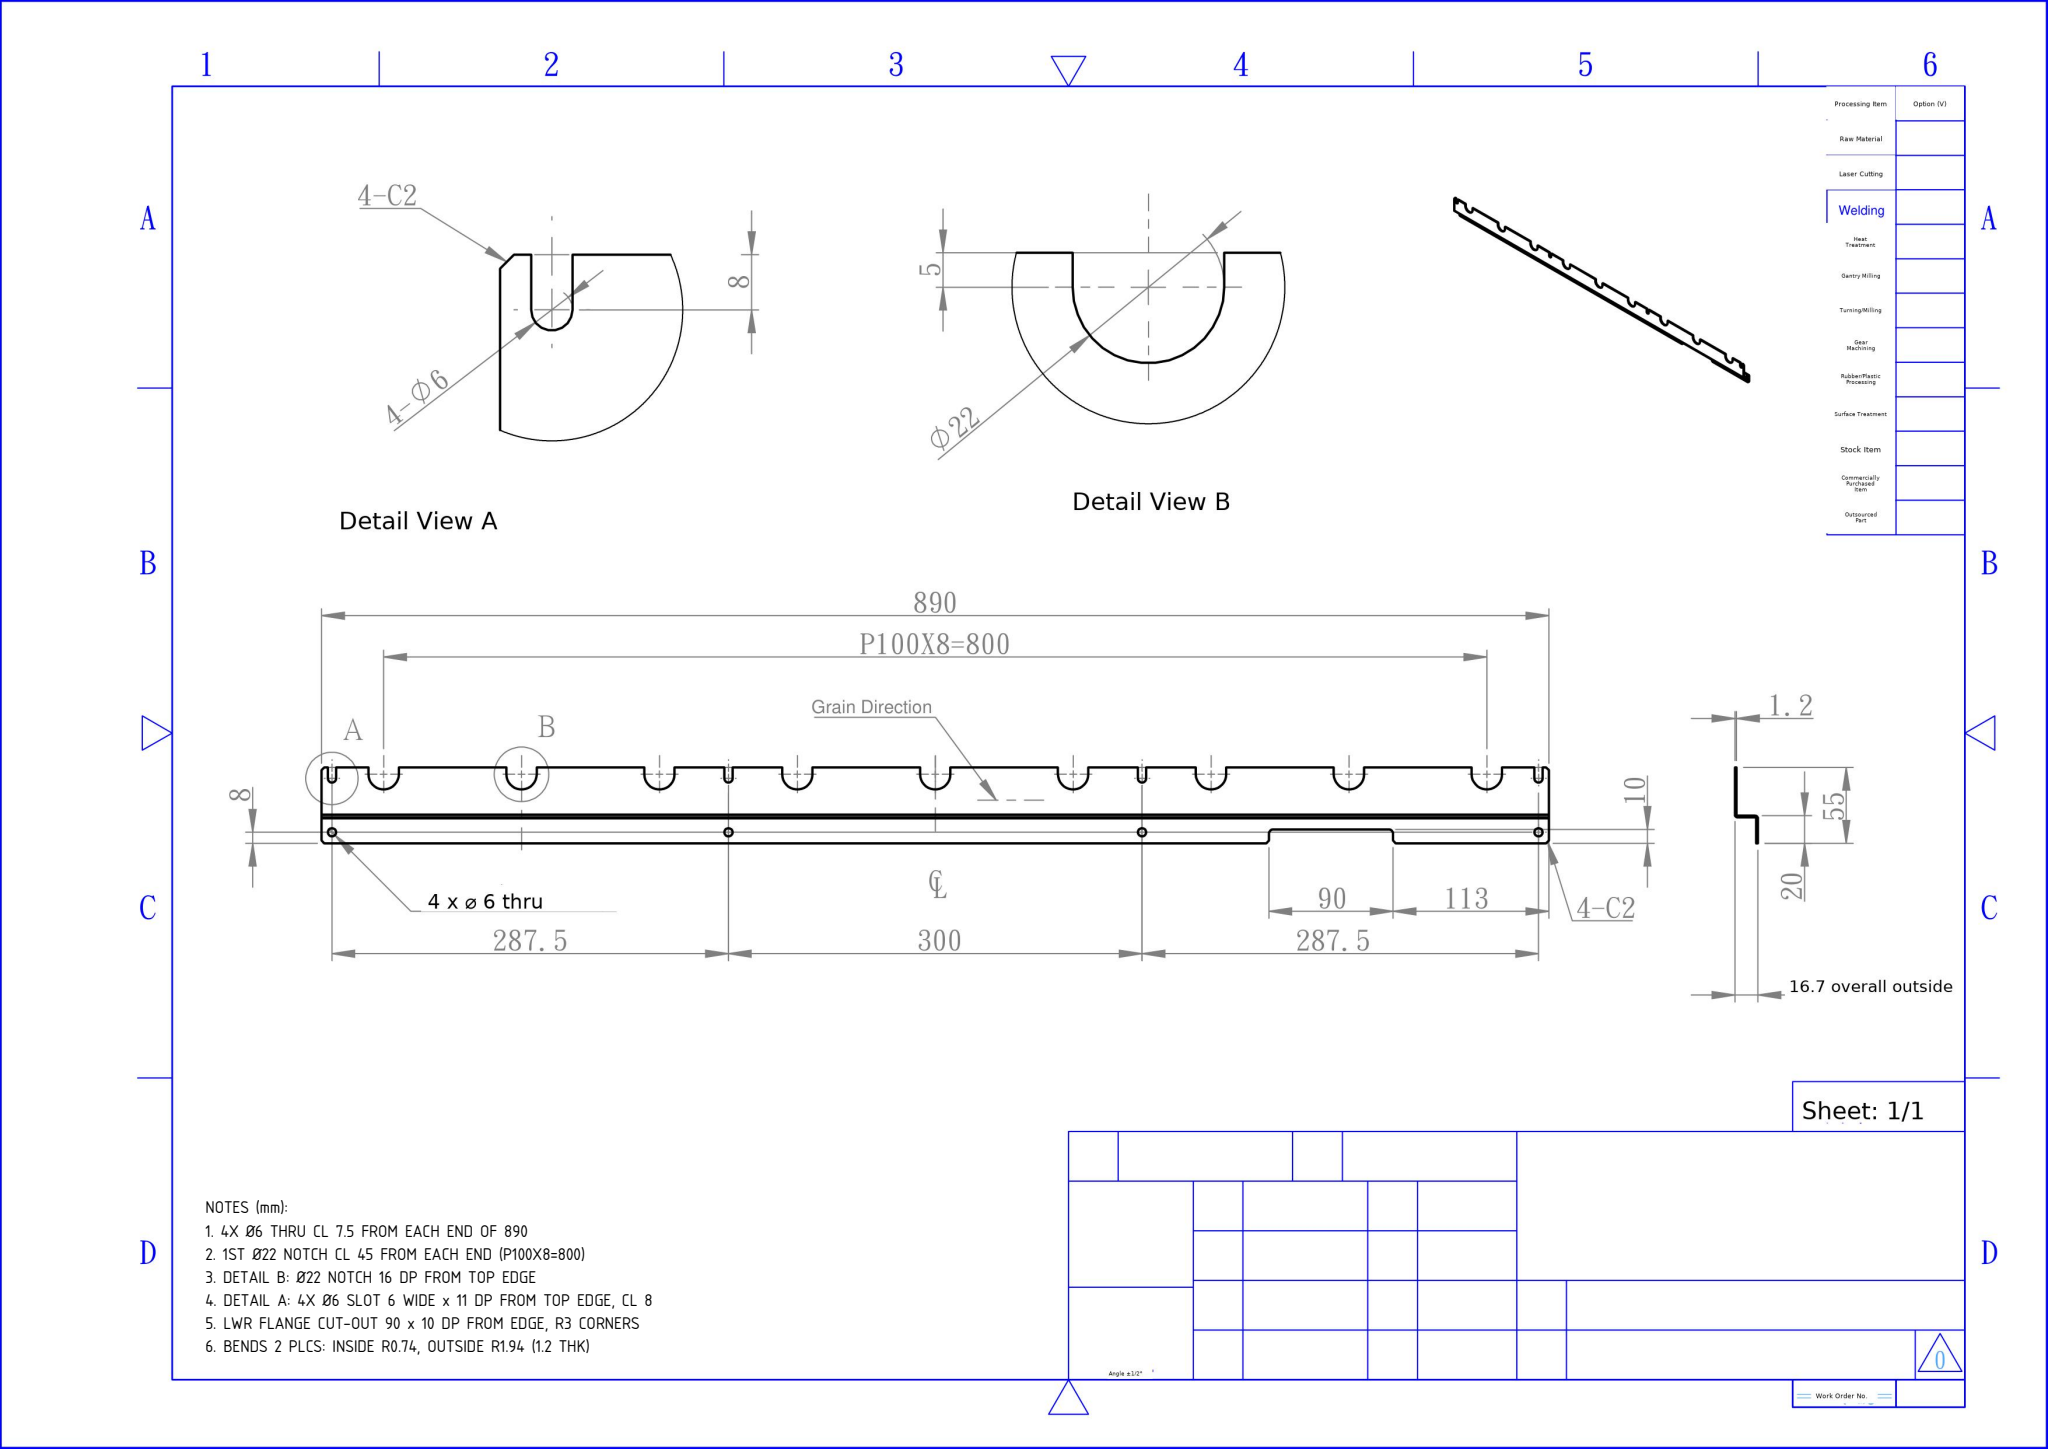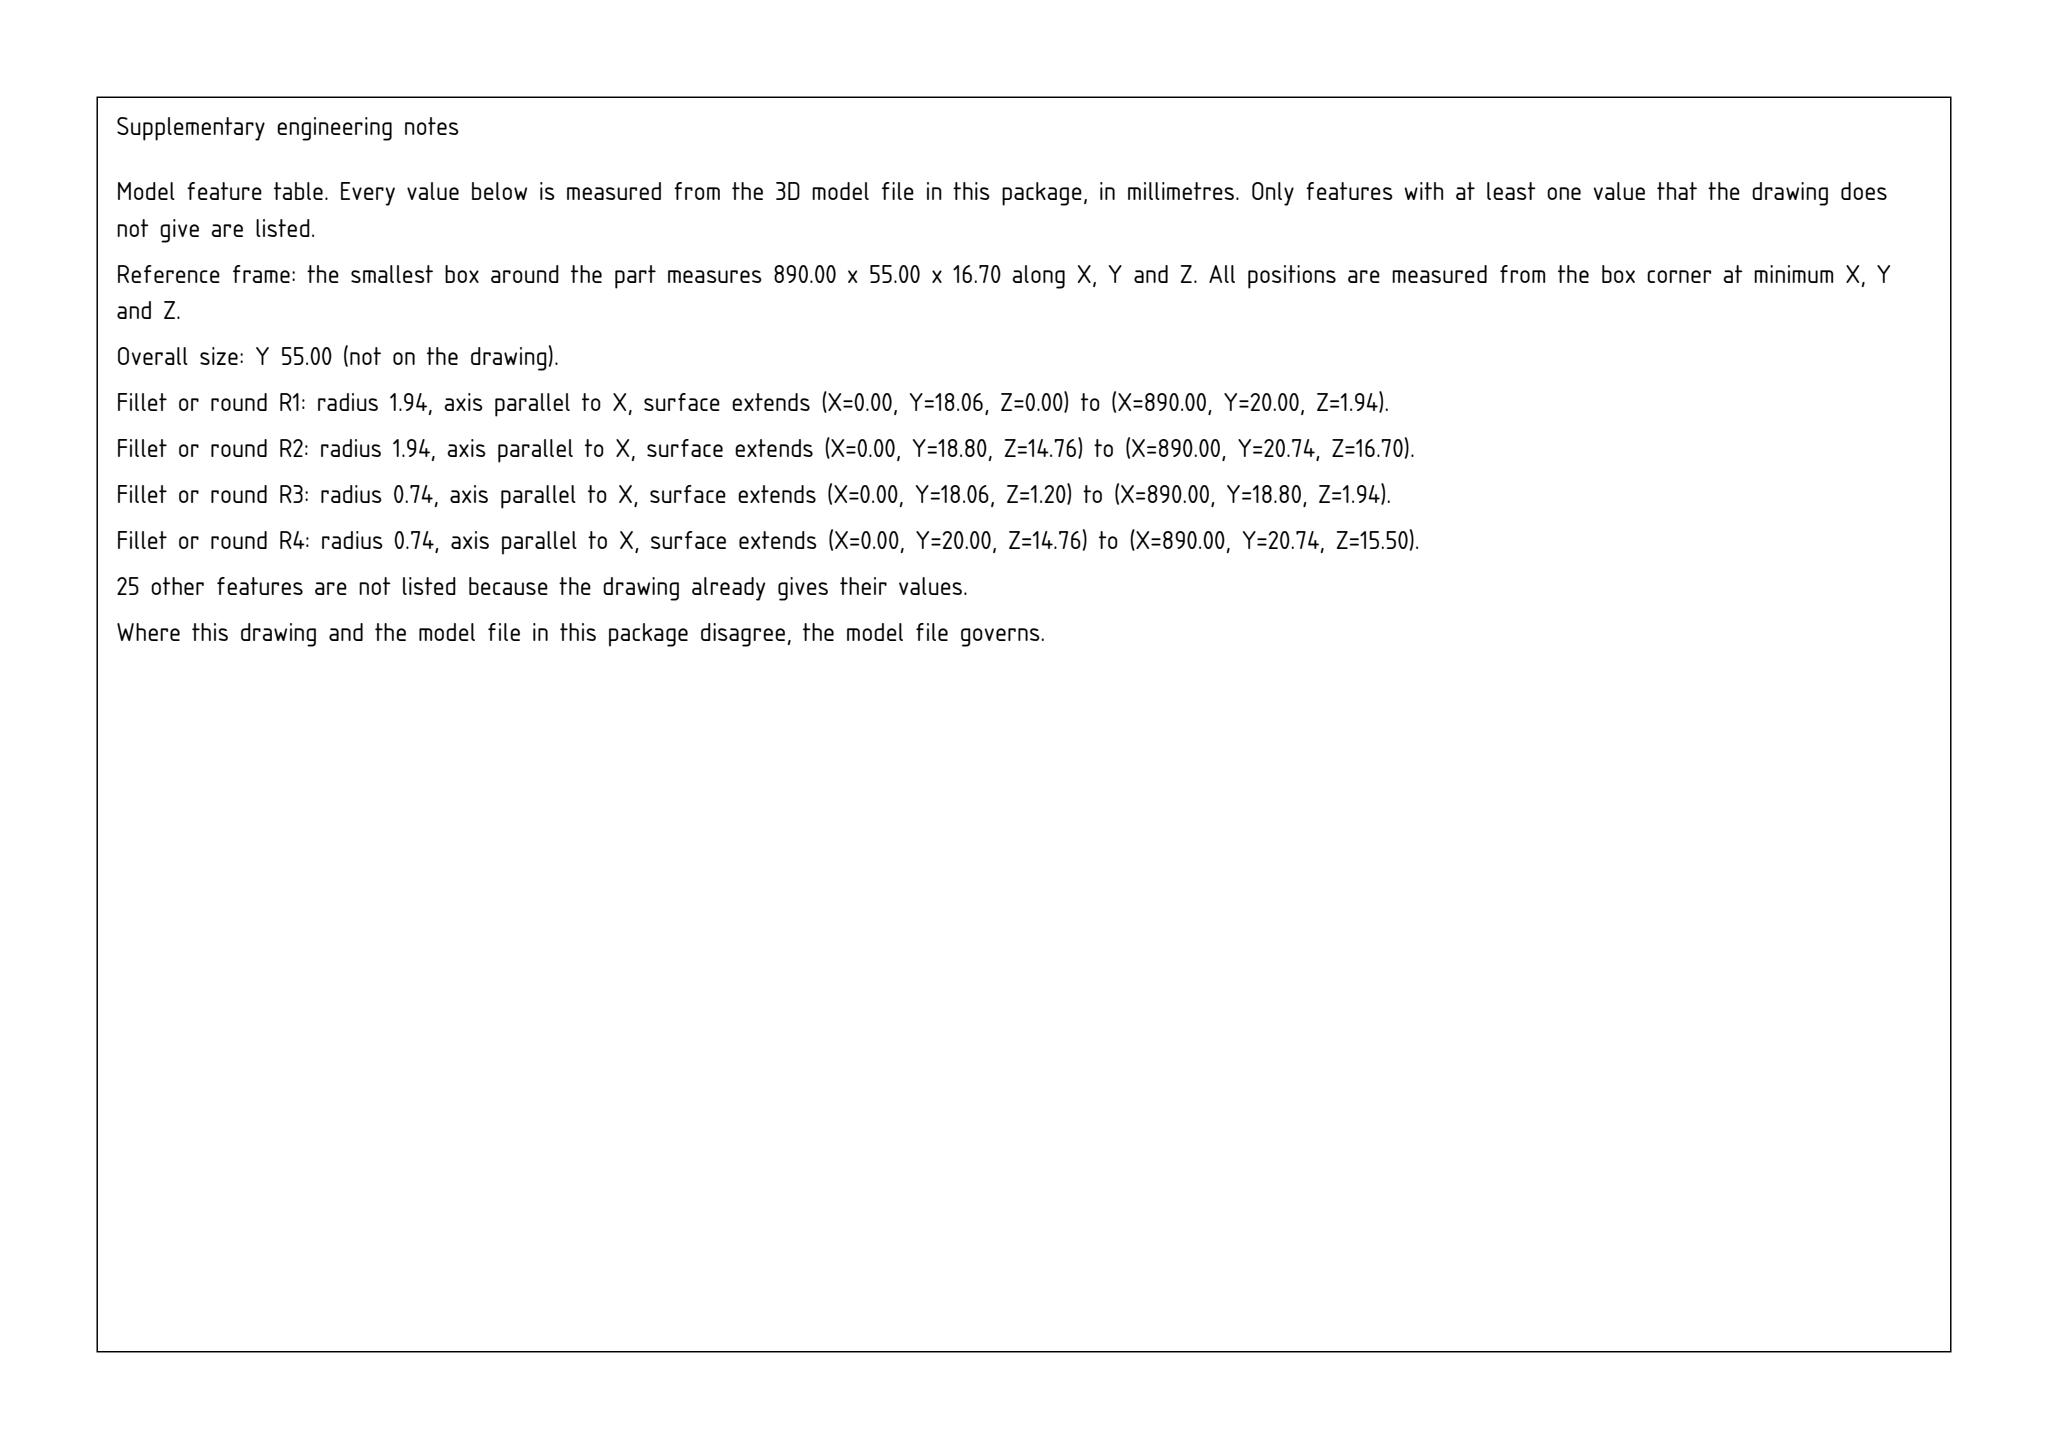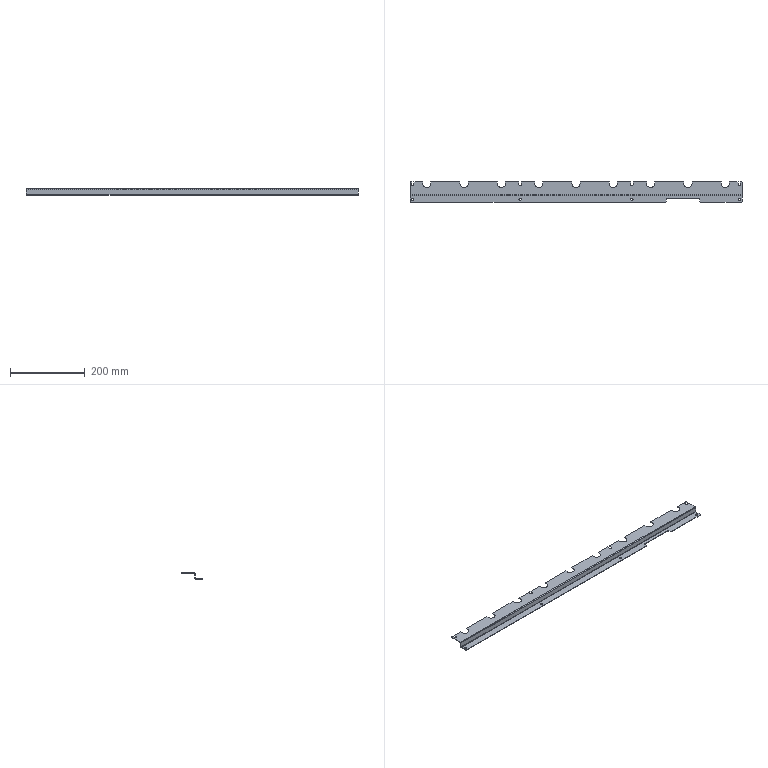Part | SolidWorks | mm | 1 solid | 94 faces | box 890 x 55 x 16.7 mm | volume 69304 mm3 | plane 67 | cylinder 27 | commonest cylinder face diameters 6 x14 22 x9 3.873 x2 1.473 x2
Drawing notes:
4X Ø6 THRU CL 7.5 FROM EACH END OF 890 | from the solid: Ø6 z-cyls y=8 at x=7.5,295,595,882.5; 890-882.5=7.5; chain 287.5/300/287.5
1ST Ø22 NOTCH CL 45 FROM EACH END (P100X8=800) | from the solid: Ø22 z-cyls at x=45,145...845; bbox x=890 -> 45 from each end, 100 pitch
DETAIL B: Ø22 NOTCH 16 DP FROM TOP EDGE | from the solid: Ø22 cyls at y=50, top edge y=55 -> CL 5; depth 5+11=16
DETAIL A: 4X Ø6 SLOT 6 WIDE x 11 DP FROM TOP EDGE, CL 8 | from the solid: Ø6 cyls y=47 at x=7.5/295/595/882.5; slot sides 4.5/10.5, 292/298, 592/598, 879.5/885.5
LWR FLANGE CUT-OUT 90 x 10 DP FROM EDGE, R3 CORNERS | from the solid: x-planes 687 & 777 (90 apart, 113 from x=890); y-plane 10 floor; Ø6 corner cyls (690,7),(774,7)
BENDS 2 PLCS: INSIDE R0.74, OUTSIDE R1.94 (1.2 THK) | from the solid: x-axis cyls dia 1.473 & 3.873 at (y18.06,z1.94) and (y20.74,z14.76); delta r = 1.2 = thk